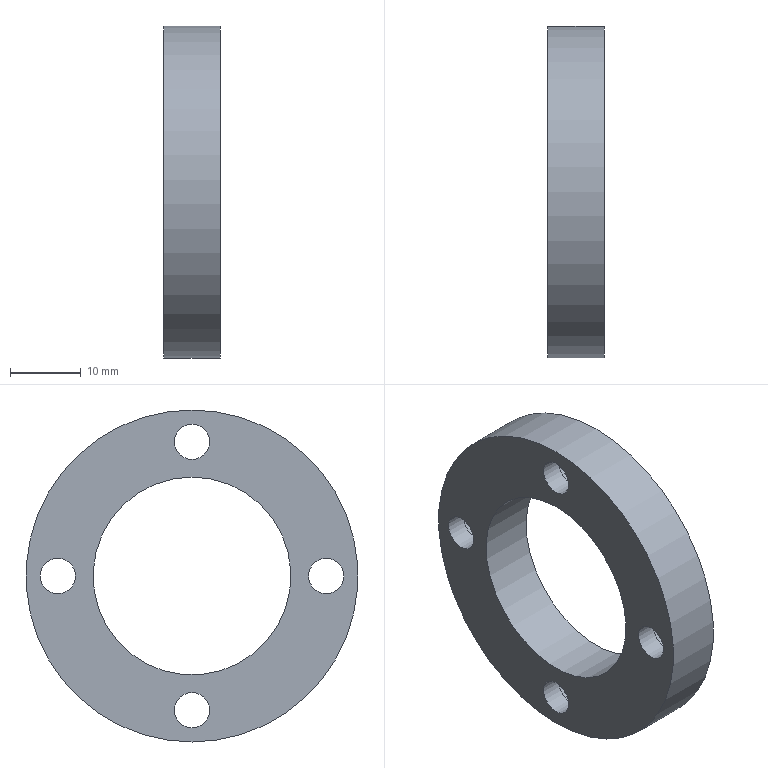Component | NX | SPACER_SLEEVE | 1 solid | 16 faces | box 8 x 47 x 47 mm | volume 7948 mm3 | cylinder 10 | plane 6 | commonest cylinder face diameters 5 x4 7 x4 47 x1 28 x1
STEP:
#1=CARTESIAN_POINT('',(0.,0.,0.));
#2=DIRECTION('',(0.,0.,1.));
#3=DIRECTION('',(1.,0.,0.));
#4=AXIS2_PLACEMENT_3D('',#1,#2,#3);
#5=CARTESIAN_POINT('',(-7.772,-17.527,-244.719));
#6=VERTEX_POINT('',#5);
#7=CARTESIAN_POINT('',(-7.772,-17.527,-258.719));
#8=DIRECTION('',(-1.,0.,0.));
#9=DIRECTION('',(0.,0.,1.));
#10=AXIS2_PLACEMENT_3D('',#7,#8,#9);
#11=CIRCLE('',#10,14.);
#12=CARTESIAN_POINT('',(-7.772,-17.527,-258.719));
#13=DIRECTION('',(1.,0.,0.));
#14=DIRECTION('',(0.,0.,-1.));
#15=AXIS2_PLACEMENT_3D('',#12,#13,#14);
#16=PLANE('',#15);
#17=CARTESIAN_POINT('',(-14.,0.));
#18=CARTESIAN_POINT('',(-14.,24.249));
#19=CARTESIAN_POINT('',(7.,12.124));
#20=CARTESIAN_POINT('',(28.,0.));
#21=CARTESIAN_POINT('',(7.,-12.124));
#22=CARTESIAN_POINT('',(-14.,-24.249));
#23=CARTESIAN_POINT('',(-14.,0.));
#24=(BOUNDED_CURVE()B_SPLINE_CURVE(2,(#17,#18,#19,#20,#21,#22,#23),.UNSPECIFIED.,.T.,.F.)B_SPLINE_CURVE_WITH_KNOTS((1,2,2,2,2,1),(-2.094,0.,2.094,4.189,6.283,8.378),.UNSPECIFIED.)CURVE()GEOMETRIC_REPRESENTATION_ITEM()RATIONAL_B_SPLINE_CURVE((1.,0.5,1.,0.5,1.,0.5,1.))REPRESENTATION_ITEM(''));
#25=(GEOMETRIC_REPRESENTATION_CONTEXT(2)PARAMETRIC_REPRESENTATION_CONTEXT()REPRESENTATION_CONTEXT('',''));
#26=DEFINITIONAL_REPRESENTATION('',(#24),#25);
#27=PCURVE('',#16,#26);
#28=CARTESIAN_POINT('',(-7.772,-17.527,-258.719));
#29=DIRECTION('',(-1.,0.,0.));
#30=DIRECTION('',(0.,0.,1.));
#31=AXIS2_PLACEMENT_3D('',#28,#29,#30);
#32=CYLINDRICAL_SURFACE('',#31,14.);
#33=CARTESIAN_POINT('',(0.,0.));
#34=DIRECTION('',(1.,0.));
#35=VECTOR('',#34,1.);
#36=LINE('',#33,#35);
#37=(GEOMETRIC_REPRESENTATION_CONTEXT(2)PARAMETRIC_REPRESENTATION_CONTEXT()REPRESENTATION_CONTEXT('',''));
#38=DEFINITIONAL_REPRESENTATION('',(#36),#37);
#39=PCURVE('',#32,#38);
#40=SURFACE_CURVE('',#11,(#27,#39),.PCURVE_S1.);
#41=EDGE_CURVE('',#6,#6,#40,.T.);
#42=ORIENTED_EDGE('',*,*,#41,.T.);
#43=EDGE_LOOP('',(#42));
#44=FACE_BOUND('',#43,.T.);
#45=CARTESIAN_POINT('',(-7.772,-17.527,-274.219));
#46=VERTEX_POINT('',#45);
#47=CARTESIAN_POINT('',(-7.772,-17.527,-277.719));
#48=DIRECTION('',(-1.,0.,0.));
#49=DIRECTION('',(0.,0.,1.));
#50=AXIS2_PLACEMENT_3D('',#47,#48,#49);
#51=CIRCLE('',#50,3.5);
#52=CARTESIAN_POINT('',(15.5,-0.));
#53=CARTESIAN_POINT('',(15.5,6.062));
#54=CARTESIAN_POINT('',(20.75,3.031));
#55=CARTESIAN_POINT('',(26.,-0.));
#56=CARTESIAN_POINT('',(20.75,-3.031));
#57=CARTESIAN_POINT('',(15.5,-6.062));
#58=CARTESIAN_POINT('',(15.5,-0.));
#59=(BOUNDED_CURVE()B_SPLINE_CURVE(2,(#52,#53,#54,#55,#56,#57,#58),.UNSPECIFIED.,.T.,.F.)B_SPLINE_CURVE_WITH_KNOTS((1,2,2,2,2,1),(-2.094,0.,2.094,4.189,6.283,8.378),.UNSPECIFIED.)CURVE()GEOMETRIC_REPRESENTATION_ITEM()RATIONAL_B_SPLINE_CURVE((1.,0.5,1.,0.5,1.,0.5,1.))REPRESENTATION_ITEM(''));
#60=(GEOMETRIC_REPRESENTATION_CONTEXT(2)PARAMETRIC_REPRESENTATION_CONTEXT()REPRESENTATION_CONTEXT('',''));
#61=DEFINITIONAL_REPRESENTATION('',(#59),#60);
#62=PCURVE('',#16,#61);
#63=CARTESIAN_POINT('',(-7.772,-17.527,-277.719));
#64=DIRECTION('',(-1.,0.,0.));
#65=DIRECTION('',(0.,0.,1.));
#66=AXIS2_PLACEMENT_3D('',#63,#64,#65);
#67=CYLINDRICAL_SURFACE('',#66,3.5);
#68=CARTESIAN_POINT('',(0.,0.));
#69=DIRECTION('',(1.,0.));
#70=VECTOR('',#69,1.);
#71=LINE('',#68,#70);
#72=(GEOMETRIC_REPRESENTATION_CONTEXT(2)PARAMETRIC_REPRESENTATION_CONTEXT()REPRESENTATION_CONTEXT('',''));
#73=DEFINITIONAL_REPRESENTATION('',(#71),#72);
#74=PCURVE('',#67,#73);
#75=SURFACE_CURVE('',#51,(#62,#74),.PCURVE_S1.);
#76=EDGE_CURVE('',#46,#46,#75,.T.);
#77=ORIENTED_EDGE('',*,*,#76,.T.);
#78=EDGE_LOOP('',(#77));
#79=FACE_BOUND('',#78,.T.);
#80=CARTESIAN_POINT('',(-7.772,-36.527,-255.219));
#81=VERTEX_POINT('',#80);
#82=CARTESIAN_POINT('',(-7.772,-36.527,-258.719));
#83=DIRECTION('',(-1.,0.,0.));
#84=DIRECTION('',(0.,0.,1.));
#85=AXIS2_PLACEMENT_3D('',#82,#83,#84);
#86=CIRCLE('',#85,3.5);
#87=CARTESIAN_POINT('',(-3.5,-19.));
#88=CARTESIAN_POINT('',(-3.5,-12.938));
#89=CARTESIAN_POINT('',(1.75,-15.969));
#90=CARTESIAN_POINT('',(7.,-19.));
#91=CARTESIAN_POINT('',(1.75,-22.031));
#92=CARTESIAN_POINT('',(-3.5,-25.062));
#93=CARTESIAN_POINT('',(-3.5,-19.));
#94=(BOUNDED_CURVE()B_SPLINE_CURVE(2,(#87,#88,#89,#90,#91,#92,#93),.UNSPECIFIED.,.T.,.F.)B_SPLINE_CURVE_WITH_KNOTS((1,2,2,2,2,1),(-2.094,0.,2.094,4.189,6.283,8.378),.UNSPECIFIED.)CURVE()GEOMETRIC_REPRESENTATION_ITEM()RATIONAL_B_SPLINE_CURVE((1.,0.5,1.,0.5,1.,0.5,1.))REPRESENTATION_ITEM(''));
#95=(GEOMETRIC_REPRESENTATION_CONTEXT(2)PARAMETRIC_REPRESENTATION_CONTEXT()REPRESENTATION_CONTEXT('',''));
#96=DEFINITIONAL_REPRESENTATION('',(#94),#95);
#97=PCURVE('',#16,#96);
#98=CARTESIAN_POINT('',(-7.772,-36.527,-258.719));
#99=DIRECTION('',(-1.,0.,0.));
#100=DIRECTION('',(0.,0.,1.));
#101=AXIS2_PLACEMENT_3D('',#98,#99,#100);
#102=CYLINDRICAL_SURFACE('',#101,3.5);
#103=CARTESIAN_POINT('',(0.,0.));
#104=DIRECTION('',(1.,0.));
#105=VECTOR('',#104,1.);
#106=LINE('',#103,#105);
#107=(GEOMETRIC_REPRESENTATION_CONTEXT(2)PARAMETRIC_REPRESENTATION_CONTEXT()REPRESENTATION_CONTEXT('',''));
#108=DEFINITIONAL_REPRESENTATION('',(#106),#107);
#109=PCURVE('',#102,#108);
#110=SURFACE_CURVE('',#86,(#97,#109),.PCURVE_S1.);
#111=EDGE_CURVE('',#81,#81,#110,.T.);
#112=ORIENTED_EDGE('',*,*,#111,.T.);
#113=EDGE_LOOP('',(#112));
#114=FACE_BOUND('',#113,.T.);
#115=CARTESIAN_POINT('',(-7.772,-17.527,-236.219));
#116=VERTEX_POINT('',#115);
#117=CARTESIAN_POINT('',(-7.772,-17.527,-239.719));
#118=DIRECTION('',(-1.,0.,0.));
#119=DIRECTION('',(0.,0.,1.));
#120=AXIS2_PLACEMENT_3D('',#117,#118,#119);
#121=CIRCLE('',#120,3.5);
#122=CARTESIAN_POINT('',(-22.5,0.));
#123=CARTESIAN_POINT('',(-22.5,6.062));
#124=CARTESIAN_POINT('',(-17.25,3.031));
#125=CARTESIAN_POINT('',(-12.,0.));
#126=CARTESIAN_POINT('',(-17.25,-3.031));
#127=CARTESIAN_POINT('',(-22.5,-6.062));
#128=CARTESIAN_POINT('',(-22.5,0.));
#129=(BOUNDED_CURVE()B_SPLINE_CURVE(2,(#122,#123,#124,#125,#126,#127,#128),.UNSPECIFIED.,.T.,.F.)B_SPLINE_CURVE_WITH_KNOTS((1,2,2,2,2,1),(-2.094,0.,2.094,4.189,6.283,8.378),.UNSPECIFIED.)CURVE()GEOMETRIC_REPRESENTATION_ITEM()RATIONAL_B_SPLINE_CURVE((1.,0.5,1.,0.5,1.,0.5,1.))REPRESENTATION_ITEM(''));
#130=(GEOMETRIC_REPRESENTATION_CONTEXT(2)PARAMETRIC_REPRESENTATION_CONTEXT()REPRESENTATION_CONTEXT('',''));
#131=DEFINITIONAL_REPRESENTATION('',(#129),#130);
#132=PCURVE('',#16,#131);
#133=CARTESIAN_POINT('',(-7.772,-17.527,-239.719));
#134=DIRECTION('',(-1.,0.,0.));
#135=DIRECTION('',(0.,0.,1.));
#136=AXIS2_PLACEMENT_3D('',#133,#134,#135);
#137=CYLINDRICAL_SURFACE('',#136,3.5);
#138=CARTESIAN_POINT('',(0.,0.));
#139=DIRECTION('',(1.,0.));
#140=VECTOR('',#139,1.);
#141=LINE('',#138,#140);
#142=(GEOMETRIC_REPRESENTATION_CONTEXT(2)PARAMETRIC_REPRESENTATION_CONTEXT()REPRESENTATION_CONTEXT('',''));
#143=DEFINITIONAL_REPRESENTATION('',(#141),#142);
#144=PCURVE('',#137,#143);
#145=SURFACE_CURVE('',#121,(#132,#144),.PCURVE_S1.);
#146=EDGE_CURVE('',#116,#116,#145,.T.);
#147=ORIENTED_EDGE('',*,*,#146,.T.);
#148=EDGE_LOOP('',(#147));
#149=FACE_BOUND('',#148,.T.);
#150=CARTESIAN_POINT('',(-7.772,1.473,-255.219));
#151=VERTEX_POINT('',#150);
#152=CARTESIAN_POINT('',(-7.772,1.473,-258.719));
#153=DIRECTION('',(-1.,0.,0.));
#154=DIRECTION('',(0.,0.,1.));
#155=AXIS2_PLACEMENT_3D('',#152,#153,#154);
#156=CIRCLE('',#155,3.5);
#157=CARTESIAN_POINT('',(-3.5,19.));
#158=CARTESIAN_POINT('',(-3.5,25.062));
#159=CARTESIAN_POINT('',(1.75,22.031));
#160=CARTESIAN_POINT('',(7.,19.));
#161=CARTESIAN_POINT('',(1.75,15.969));
#162=CARTESIAN_POINT('',(-3.5,12.938));
#163=CARTESIAN_POINT('',(-3.5,19.));
#164=(BOUNDED_CURVE()B_SPLINE_CURVE(2,(#157,#158,#159,#160,#161,#162,#163),.UNSPECIFIED.,.T.,.F.)B_SPLINE_CURVE_WITH_KNOTS((1,2,2,2,2,1),(-2.094,0.,2.094,4.189,6.283,8.378),.UNSPECIFIED.)CURVE()GEOMETRIC_REPRESENTATION_ITEM()RATIONAL_B_SPLINE_CURVE((1.,0.5,1.,0.5,1.,0.5,1.))REPRESENTATION_ITEM(''));
#165=(GEOMETRIC_REPRESENTATION_CONTEXT(2)PARAMETRIC_REPRESENTATION_CONTEXT()REPRESENTATION_CONTEXT('',''));
#166=DEFINITIONAL_REPRESENTATION('',(#164),#165);
#167=PCURVE('',#16,#166);
#168=CARTESIAN_POINT('',(-7.772,1.473,-258.719));
#169=DIRECTION('',(-1.,0.,0.));
#170=DIRECTION('',(0.,0.,1.));
#171=AXIS2_PLACEMENT_3D('',#168,#169,#170);
#172=CYLINDRICAL_SURFACE('',#171,3.5);
#173=CARTESIAN_POINT('',(0.,0.));
#174=DIRECTION('',(1.,0.));
#175=VECTOR('',#174,1.);
#176=LINE('',#173,#175);
#177=(GEOMETRIC_REPRESENTATION_CONTEXT(2)PARAMETRIC_REPRESENTATION_CONTEXT()REPRESENTATION_CONTEXT('',''));
#178=DEFINITIONAL_REPRESENTATION('',(#176),#177);
#179=PCURVE('',#172,#178);
#180=SURFACE_CURVE('',#156,(#167,#179),.PCURVE_S1.);
#181=EDGE_CURVE('',#151,#151,#180,.T.);
#182=ORIENTED_EDGE('',*,*,#181,.T.);
#183=EDGE_LOOP('',(#182));
#184=FACE_BOUND('',#183,.T.);
#185=CARTESIAN_POINT('',(-7.772,-17.527,-282.219));
#186=VERTEX_POINT('',#185);
#187=CARTESIAN_POINT('',(-7.772,-17.527,-258.719));
#188=DIRECTION('',(-1.,0.,0.));
#189=DIRECTION('',(0.,0.,-1.));
#190=AXIS2_PLACEMENT_3D('',#187,#188,#189);
#191=CIRCLE('',#190,23.5);
#192=CARTESIAN_POINT('',(23.5,0.));
#193=CARTESIAN_POINT('',(23.5,-40.703));
#194=CARTESIAN_POINT('',(-11.75,-20.352));
#195=CARTESIAN_POINT('',(-47.,-0.));
#196=CARTESIAN_POINT('',(-11.75,20.352));
#197=CARTESIAN_POINT('',(23.5,40.703));
#198=CARTESIAN_POINT('',(23.5,0.));
#199=(BOUNDED_CURVE()B_SPLINE_CURVE(2,(#192,#193,#194,#195,#196,#197,#198),.UNSPECIFIED.,.T.,.F.)B_SPLINE_CURVE_WITH_KNOTS((1,2,2,2,2,1),(-2.094,0.,2.094,4.189,6.283,8.378),.UNSPECIFIED.)CURVE()GEOMETRIC_REPRESENTATION_ITEM()RATIONAL_B_SPLINE_CURVE((1.,0.5,1.,0.5,1.,0.5,1.))REPRESENTATION_ITEM(''));
#200=(GEOMETRIC_REPRESENTATION_CONTEXT(2)PARAMETRIC_REPRESENTATION_CONTEXT()REPRESENTATION_CONTEXT('',''));
#201=DEFINITIONAL_REPRESENTATION('',(#199),#200);
#202=PCURVE('',#16,#201);
#203=CARTESIAN_POINT('',(-15.772,-17.527,-258.719));
#204=DIRECTION('',(1.,0.,0.));
#205=DIRECTION('',(0.,0.,-1.));
#206=AXIS2_PLACEMENT_3D('',#203,#204,#205);
#207=CYLINDRICAL_SURFACE('',#206,23.5);
#208=CARTESIAN_POINT('',(6.283,8.));
#209=DIRECTION('',(-1.,0.));
#210=VECTOR('',#209,1.);
#211=LINE('',#208,#210);
#212=(GEOMETRIC_REPRESENTATION_CONTEXT(2)PARAMETRIC_REPRESENTATION_CONTEXT()REPRESENTATION_CONTEXT('',''));
#213=DEFINITIONAL_REPRESENTATION('',(#211),#212);
#214=PCURVE('',#207,#213);
#215=SURFACE_CURVE('',#191,(#202,#214),.PCURVE_S1.);
#216=EDGE_CURVE('',#186,#186,#215,.T.);
#217=ORIENTED_EDGE('',*,*,#216,.F.);
#218=EDGE_LOOP('',(#217));
#219=FACE_BOUND('',#218,.T.);
#220=ADVANCED_FACE('',(#44,#79,#114,#149,#184,#219),#16,.T.);
#221=CARTESIAN_POINT('',(-15.772,-17.527,-244.719));
#222=VERTEX_POINT('',#221);
#223=CARTESIAN_POINT('',(-15.772,-17.527,-258.719));
#224=DIRECTION('',(-1.,0.,0.));
#225=DIRECTION('',(0.,0.,1.));
#226=AXIS2_PLACEMENT_3D('',#223,#224,#225);
#227=CIRCLE('',#226,14.);
#228=CARTESIAN_POINT('',(-15.772,-17.527,-258.719));
#229=DIRECTION('',(-1.,0.,0.));
#230=DIRECTION('',(0.,0.,1.));
#231=AXIS2_PLACEMENT_3D('',#228,#229,#230);
#232=PLANE('',#231);
#233=CARTESIAN_POINT('',(0.,0.));
#234=DIRECTION('',(1.,0.));
#235=AXIS2_PLACEMENT_2D('',#233,#234);
#236=CIRCLE('',#235,14.);
#237=(GEOMETRIC_REPRESENTATION_CONTEXT(2)PARAMETRIC_REPRESENTATION_CONTEXT()REPRESENTATION_CONTEXT('',''));
#238=DEFINITIONAL_REPRESENTATION('',(#236),#237);
#239=PCURVE('',#232,#238);
#240=CARTESIAN_POINT('',(0.,8.));
#241=DIRECTION('',(1.,0.));
#242=VECTOR('',#241,1.);
#243=LINE('',#240,#242);
#244=(GEOMETRIC_REPRESENTATION_CONTEXT(2)PARAMETRIC_REPRESENTATION_CONTEXT()REPRESENTATION_CONTEXT('',''));
#245=DEFINITIONAL_REPRESENTATION('',(#243),#244);
#246=PCURVE('',#32,#245);
#247=SURFACE_CURVE('',#227,(#239,#246),.PCURVE_S1.);
#248=EDGE_CURVE('',#222,#222,#247,.T.);
#249=ORIENTED_EDGE('',*,*,#248,.F.);
#250=EDGE_LOOP('',(#249));
#251=FACE_BOUND('',#250,.T.);
#252=CARTESIAN_POINT('',(-15.772,-17.527,-275.219));
#253=VERTEX_POINT('',#252);
#254=CARTESIAN_POINT('',(-15.772,-17.527,-277.719));
#255=DIRECTION('',(-1.,0.,0.));
#256=DIRECTION('',(0.,0.,1.));
#257=AXIS2_PLACEMENT_3D('',#254,#255,#256);
#258=CIRCLE('',#257,2.5);
#259=CARTESIAN_POINT('',(-19.,-0.));
#260=DIRECTION('',(1.,0.));
#261=AXIS2_PLACEMENT_2D('',#259,#260);
#262=CIRCLE('',#261,2.5);
#263=(GEOMETRIC_REPRESENTATION_CONTEXT(2)PARAMETRIC_REPRESENTATION_CONTEXT()REPRESENTATION_CONTEXT('',''));
#264=DEFINITIONAL_REPRESENTATION('',(#262),#263);
#265=PCURVE('',#232,#264);
#266=CARTESIAN_POINT('',(-43.312,-17.527,-277.719));
#267=DIRECTION('',(-1.,0.,0.));
#268=DIRECTION('',(0.,0.,1.));
#269=AXIS2_PLACEMENT_3D('',#266,#267,#268);
#270=CYLINDRICAL_SURFACE('',#269,2.5);
#271=CARTESIAN_POINT('',(0.,-27.541));
#272=DIRECTION('',(1.,0.));
#273=VECTOR('',#272,1.);
#274=LINE('',#271,#273);
#275=(GEOMETRIC_REPRESENTATION_CONTEXT(2)PARAMETRIC_REPRESENTATION_CONTEXT()REPRESENTATION_CONTEXT('',''));
#276=DEFINITIONAL_REPRESENTATION('',(#274),#275);
#277=PCURVE('',#270,#276);
#278=SURFACE_CURVE('',#258,(#265,#277),.PCURVE_S1.);
#279=EDGE_CURVE('',#253,#253,#278,.T.);
#280=ORIENTED_EDGE('',*,*,#279,.F.);
#281=EDGE_LOOP('',(#280));
#282=FACE_BOUND('',#281,.T.);
#283=CARTESIAN_POINT('',(-15.772,-36.527,-256.219));
#284=VERTEX_POINT('',#283);
#285=CARTESIAN_POINT('',(-15.772,-36.527,-258.719));
#286=DIRECTION('',(-1.,0.,0.));
#287=DIRECTION('',(0.,0.,1.));
#288=AXIS2_PLACEMENT_3D('',#285,#286,#287);
#289=CIRCLE('',#288,2.5);
#290=CARTESIAN_POINT('',(0.,-19.));
#291=DIRECTION('',(1.,0.));
#292=AXIS2_PLACEMENT_2D('',#290,#291);
#293=CIRCLE('',#292,2.5);
#294=(GEOMETRIC_REPRESENTATION_CONTEXT(2)PARAMETRIC_REPRESENTATION_CONTEXT()REPRESENTATION_CONTEXT('',''));
#295=DEFINITIONAL_REPRESENTATION('',(#293),#294);
#296=PCURVE('',#232,#295);
#297=CARTESIAN_POINT('',(-43.312,-36.527,-258.719));
#298=DIRECTION('',(-1.,0.,0.));
#299=DIRECTION('',(0.,0.,1.));
#300=AXIS2_PLACEMENT_3D('',#297,#298,#299);
#301=CYLINDRICAL_SURFACE('',#300,2.5);
#302=CARTESIAN_POINT('',(0.,-27.541));
#303=DIRECTION('',(1.,0.));
#304=VECTOR('',#303,1.);
#305=LINE('',#302,#304);
#306=(GEOMETRIC_REPRESENTATION_CONTEXT(2)PARAMETRIC_REPRESENTATION_CONTEXT()REPRESENTATION_CONTEXT('',''));
#307=DEFINITIONAL_REPRESENTATION('',(#305),#306);
#308=PCURVE('',#301,#307);
#309=SURFACE_CURVE('',#289,(#296,#308),.PCURVE_S1.);
#310=EDGE_CURVE('',#284,#284,#309,.T.);
#311=ORIENTED_EDGE('',*,*,#310,.F.);
#312=EDGE_LOOP('',(#311));
#313=FACE_BOUND('',#312,.T.);
#314=CARTESIAN_POINT('',(-15.772,-17.527,-237.219));
#315=VERTEX_POINT('',#314);
#316=CARTESIAN_POINT('',(-15.772,-17.527,-239.719));
#317=DIRECTION('',(-1.,0.,0.));
#318=DIRECTION('',(0.,0.,1.));
#319=AXIS2_PLACEMENT_3D('',#316,#317,#318);
#320=CIRCLE('',#319,2.5);
#321=CARTESIAN_POINT('',(19.,0.));
#322=DIRECTION('',(1.,0.));
#323=AXIS2_PLACEMENT_2D('',#321,#322);
#324=CIRCLE('',#323,2.5);
#325=(GEOMETRIC_REPRESENTATION_CONTEXT(2)PARAMETRIC_REPRESENTATION_CONTEXT()REPRESENTATION_CONTEXT('',''));
#326=DEFINITIONAL_REPRESENTATION('',(#324),#325);
#327=PCURVE('',#232,#326);
#328=CARTESIAN_POINT('',(-43.312,-17.527,-239.719));
#329=DIRECTION('',(-1.,0.,0.));
#330=DIRECTION('',(0.,0.,1.));
#331=AXIS2_PLACEMENT_3D('',#328,#329,#330);
#332=CYLINDRICAL_SURFACE('',#331,2.5);
#333=CARTESIAN_POINT('',(0.,-27.541));
#334=DIRECTION('',(1.,0.));
#335=VECTOR('',#334,1.);
#336=LINE('',#333,#335);
#337=(GEOMETRIC_REPRESENTATION_CONTEXT(2)PARAMETRIC_REPRESENTATION_CONTEXT()REPRESENTATION_CONTEXT('',''));
#338=DEFINITIONAL_REPRESENTATION('',(#336),#337);
#339=PCURVE('',#332,#338);
#340=SURFACE_CURVE('',#320,(#327,#339),.PCURVE_S1.);
#341=EDGE_CURVE('',#315,#315,#340,.T.);
#342=ORIENTED_EDGE('',*,*,#341,.F.);
#343=EDGE_LOOP('',(#342));
#344=FACE_BOUND('',#343,.T.);
#345=CARTESIAN_POINT('',(-15.772,1.473,-256.219));
#346=VERTEX_POINT('',#345);
#347=CARTESIAN_POINT('',(-15.772,1.473,-258.719));
#348=DIRECTION('',(-1.,0.,0.));
#349=DIRECTION('',(0.,0.,1.));
#350=AXIS2_PLACEMENT_3D('',#347,#348,#349);
#351=CIRCLE('',#350,2.5);
#352=CARTESIAN_POINT('',(-0.,19.));
#353=DIRECTION('',(1.,0.));
#354=AXIS2_PLACEMENT_2D('',#352,#353);
#355=CIRCLE('',#354,2.5);
#356=(GEOMETRIC_REPRESENTATION_CONTEXT(2)PARAMETRIC_REPRESENTATION_CONTEXT()REPRESENTATION_CONTEXT('',''));
#357=DEFINITIONAL_REPRESENTATION('',(#355),#356);
#358=PCURVE('',#232,#357);
#359=CARTESIAN_POINT('',(-43.312,1.473,-258.719));
#360=DIRECTION('',(-1.,0.,0.));
#361=DIRECTION('',(0.,0.,1.));
#362=AXIS2_PLACEMENT_3D('',#359,#360,#361);
#363=CYLINDRICAL_SURFACE('',#362,2.5);
#364=CARTESIAN_POINT('',(0.,-27.541));
#365=DIRECTION('',(1.,0.));
#366=VECTOR('',#365,1.);
#367=LINE('',#364,#366);
#368=(GEOMETRIC_REPRESENTATION_CONTEXT(2)PARAMETRIC_REPRESENTATION_CONTEXT()REPRESENTATION_CONTEXT('',''));
#369=DEFINITIONAL_REPRESENTATION('',(#367),#368);
#370=PCURVE('',#363,#369);
#371=SURFACE_CURVE('',#351,(#358,#370),.PCURVE_S1.);
#372=EDGE_CURVE('',#346,#346,#371,.T.);
#373=ORIENTED_EDGE('',*,*,#372,.F.);
#374=EDGE_LOOP('',(#373));
#375=FACE_BOUND('',#374,.T.);
#376=CARTESIAN_POINT('',(-15.772,-17.527,-282.219));
#377=VERTEX_POINT('',#376);
#378=CARTESIAN_POINT('',(-15.772,-17.527,-258.719));
#379=DIRECTION('',(1.,0.,0.));
#380=DIRECTION('',(0.,0.,-1.));
#381=AXIS2_PLACEMENT_3D('',#378,#379,#380);
#382=CIRCLE('',#381,23.5);
#383=CARTESIAN_POINT('',(-23.5,0.));
#384=CARTESIAN_POINT('',(-23.5,40.703));
#385=CARTESIAN_POINT('',(11.75,20.352));
#386=CARTESIAN_POINT('',(47.,0.));
#387=CARTESIAN_POINT('',(11.75,-20.352));
#388=CARTESIAN_POINT('',(-23.5,-40.703));
#389=CARTESIAN_POINT('',(-23.5,0.));
#390=(BOUNDED_CURVE()B_SPLINE_CURVE(2,(#383,#384,#385,#386,#387,#388,#389),.UNSPECIFIED.,.T.,.F.)B_SPLINE_CURVE_WITH_KNOTS((1,2,2,2,2,1),(-2.094,0.,2.094,4.189,6.283,8.378),.UNSPECIFIED.)CURVE()GEOMETRIC_REPRESENTATION_ITEM()RATIONAL_B_SPLINE_CURVE((1.,0.5,1.,0.5,1.,0.5,1.))REPRESENTATION_ITEM(''));
#391=(GEOMETRIC_REPRESENTATION_CONTEXT(2)PARAMETRIC_REPRESENTATION_CONTEXT()REPRESENTATION_CONTEXT('',''));
#392=DEFINITIONAL_REPRESENTATION('',(#390),#391);
#393=PCURVE('',#232,#392);
#394=CARTESIAN_POINT('',(0.,0.));
#395=DIRECTION('',(1.,0.));
#396=VECTOR('',#395,1.);
#397=LINE('',#394,#396);
#398=(GEOMETRIC_REPRESENTATION_CONTEXT(2)PARAMETRIC_REPRESENTATION_CONTEXT()REPRESENTATION_CONTEXT('',''));
#399=DEFINITIONAL_REPRESENTATION('',(#397),#398);
#400=PCURVE('',#207,#399);
#401=SURFACE_CURVE('',#382,(#393,#400),.PCURVE_S1.);
#402=EDGE_CURVE('',#377,#377,#401,.T.);
#403=ORIENTED_EDGE('',*,*,#402,.F.);
#404=EDGE_LOOP('',(#403));
#405=FACE_BOUND('',#404,.T.);
#406=ADVANCED_FACE('',(#251,#282,#313,#344,#375,#405),#232,.T.);
#407=ORIENTED_EDGE('',*,*,#216,.T.);
#408=CARTESIAN_POINT('',(-15.772,-17.527,-282.219));
#409=CARTESIAN_POINT('',(-7.772,-17.527,-282.219));
#410=B_SPLINE_CURVE_WITH_KNOTS('',1,(#408,#409),.UNSPECIFIED.,.F.,.F.,(2,2),(0.,8.),.PIECEWISE_BEZIER_KNOTS.);
#411=CARTESIAN_POINT('',(0.,0.));
#412=DIRECTION('',(0.,1.));
#413=VECTOR('',#412,1.);
#414=LINE('',#411,#413);
#415=(GEOMETRIC_REPRESENTATION_CONTEXT(2)PARAMETRIC_REPRESENTATION_CONTEXT()REPRESENTATION_CONTEXT('',''));
#416=DEFINITIONAL_REPRESENTATION('',(#414),#415);
#417=PCURVE('',#207,#416);
#418=CARTESIAN_POINT('',(6.283,0.));
#419=DIRECTION('',(0.,1.));
#420=VECTOR('',#419,1.);
#421=LINE('',#418,#420);
#422=(GEOMETRIC_REPRESENTATION_CONTEXT(2)PARAMETRIC_REPRESENTATION_CONTEXT()REPRESENTATION_CONTEXT('',''));
#423=DEFINITIONAL_REPRESENTATION('',(#421),#422);
#424=PCURVE('',#207,#423);
#425=SEAM_CURVE('',#410,(#417,#424),.PCURVE_S1.);
#426=EDGE_CURVE('',#377,#186,#425,.T.);
#427=ORIENTED_EDGE('',*,*,#426,.F.);
#428=ORIENTED_EDGE('',*,*,#402,.T.);
#429=ORIENTED_EDGE('',*,*,#426,.T.);
#430=EDGE_LOOP('',(#407,#427,#428,#429));
#431=FACE_BOUND('',#430,.T.);
#432=ADVANCED_FACE('',(#431),#207,.T.);
#433=ORIENTED_EDGE('',*,*,#372,.F.);
#434=CARTESIAN_POINT('',(-12.772,1.473,-256.219));
#435=VERTEX_POINT('',#434);
#436=CARTESIAN_POINT('',(-12.772,1.473,-256.219));
#437=CARTESIAN_POINT('',(-15.772,1.473,-256.219));
#438=B_SPLINE_CURVE_WITH_KNOTS('',1,(#436,#437),.UNSPECIFIED.,.F.,.F.,(2,2),(-30.541,-27.541),.PIECEWISE_BEZIER_KNOTS.);
#439=CARTESIAN_POINT('',(0.,0.));
#440=DIRECTION('',(0.,1.));
#441=VECTOR('',#440,1.);
#442=LINE('',#439,#441);
#443=(GEOMETRIC_REPRESENTATION_CONTEXT(2)PARAMETRIC_REPRESENTATION_CONTEXT()REPRESENTATION_CONTEXT('',''));
#444=DEFINITIONAL_REPRESENTATION('',(#442),#443);
#445=PCURVE('',#363,#444);
#446=CARTESIAN_POINT('',(6.283,0.));
#447=DIRECTION('',(0.,1.));
#448=VECTOR('',#447,1.);
#449=LINE('',#446,#448);
#450=(GEOMETRIC_REPRESENTATION_CONTEXT(2)PARAMETRIC_REPRESENTATION_CONTEXT()REPRESENTATION_CONTEXT('',''));
#451=DEFINITIONAL_REPRESENTATION('',(#449),#450);
#452=PCURVE('',#363,#451);
#453=SEAM_CURVE('',#438,(#445,#452),.PCURVE_S1.);
#454=EDGE_CURVE('',#435,#346,#453,.T.);
#455=ORIENTED_EDGE('',*,*,#454,.F.);
#456=CARTESIAN_POINT('',(-12.772,1.473,-258.719));
#457=DIRECTION('',(1.,0.,0.));
#458=DIRECTION('',(0.,0.,1.));
#459=AXIS2_PLACEMENT_3D('',#456,#457,#458);
#460=CIRCLE('',#459,2.5);
#461=CARTESIAN_POINT('',(6.283,-30.541));
#462=DIRECTION('',(-1.,0.));
#463=VECTOR('',#462,1.);
#464=LINE('',#461,#463);
#465=(GEOMETRIC_REPRESENTATION_CONTEXT(2)PARAMETRIC_REPRESENTATION_CONTEXT()REPRESENTATION_CONTEXT('',''));
#466=DEFINITIONAL_REPRESENTATION('',(#464),#465);
#467=PCURVE('',#363,#466);
#468=CARTESIAN_POINT('',(-12.772,1.473,-258.719));
#469=DIRECTION('',(-1.,0.,0.));
#470=DIRECTION('',(0.,0.,1.));
#471=AXIS2_PLACEMENT_3D('',#468,#469,#470);
#472=PLANE('',#471);
#473=CARTESIAN_POINT('',(2.5,0.));
#474=CARTESIAN_POINT('',(2.5,-4.33));
#475=CARTESIAN_POINT('',(-1.25,-2.165));
#476=CARTESIAN_POINT('',(-5.,-0.));
#477=CARTESIAN_POINT('',(-1.25,2.165));
#478=CARTESIAN_POINT('',(2.5,4.33));
#479=CARTESIAN_POINT('',(2.5,0.));
#480=(BOUNDED_CURVE()B_SPLINE_CURVE(2,(#473,#474,#475,#476,#477,#478,#479),.UNSPECIFIED.,.T.,.F.)B_SPLINE_CURVE_WITH_KNOTS((1,2,2,2,2,1),(-2.094,0.,2.094,4.189,6.283,8.378),.UNSPECIFIED.)CURVE()GEOMETRIC_REPRESENTATION_ITEM()RATIONAL_B_SPLINE_CURVE((1.,0.5,1.,0.5,1.,0.5,1.))REPRESENTATION_ITEM(''));
#481=(GEOMETRIC_REPRESENTATION_CONTEXT(2)PARAMETRIC_REPRESENTATION_CONTEXT()REPRESENTATION_CONTEXT('',''));
#482=DEFINITIONAL_REPRESENTATION('',(#480),#481);
#483=PCURVE('',#472,#482);
#484=SURFACE_CURVE('',#460,(#467,#483),.PCURVE_S1.);
#485=EDGE_CURVE('',#435,#435,#484,.T.);
#486=ORIENTED_EDGE('',*,*,#485,.F.);
#487=ORIENTED_EDGE('',*,*,#454,.T.);
#488=EDGE_LOOP('',(#433,#455,#486,#487));
#489=FACE_BOUND('',#488,.F.);
#490=ADVANCED_FACE('',(#489),#363,.F.);
#491=ORIENTED_EDGE('',*,*,#485,.F.);
#492=EDGE_LOOP('',(#491));
#493=FACE_BOUND('',#492,.T.);
#494=CARTESIAN_POINT('',(-12.772,1.473,-255.219));
#495=VERTEX_POINT('',#494);
#496=CARTESIAN_POINT('',(-12.772,1.473,-258.719));
#497=DIRECTION('',(1.,0.,0.));
#498=DIRECTION('',(0.,0.,1.));
#499=AXIS2_PLACEMENT_3D('',#496,#497,#498);
#500=CIRCLE('',#499,3.5);
#501=CARTESIAN_POINT('',(3.5,0.));
#502=CARTESIAN_POINT('',(3.5,-6.062));
#503=CARTESIAN_POINT('',(-1.75,-3.031));
#504=CARTESIAN_POINT('',(-7.,-0.));
#505=CARTESIAN_POINT('',(-1.75,3.031));
#506=CARTESIAN_POINT('',(3.5,6.062));
#507=CARTESIAN_POINT('',(3.5,0.));
#508=(BOUNDED_CURVE()B_SPLINE_CURVE(2,(#501,#502,#503,#504,#505,#506,#507),.UNSPECIFIED.,.T.,.F.)B_SPLINE_CURVE_WITH_KNOTS((1,2,2,2,2,1),(-2.094,0.,2.094,4.189,6.283,8.378),.UNSPECIFIED.)CURVE()GEOMETRIC_REPRESENTATION_ITEM()RATIONAL_B_SPLINE_CURVE((1.,0.5,1.,0.5,1.,0.5,1.))REPRESENTATION_ITEM(''));
#509=(GEOMETRIC_REPRESENTATION_CONTEXT(2)PARAMETRIC_REPRESENTATION_CONTEXT()REPRESENTATION_CONTEXT('',''));
#510=DEFINITIONAL_REPRESENTATION('',(#508),#509);
#511=PCURVE('',#472,#510);
#512=CARTESIAN_POINT('',(6.283,5.));
#513=DIRECTION('',(-1.,0.));
#514=VECTOR('',#513,1.);
#515=LINE('',#512,#514);
#516=(GEOMETRIC_REPRESENTATION_CONTEXT(2)PARAMETRIC_REPRESENTATION_CONTEXT()REPRESENTATION_CONTEXT('',''));
#517=DEFINITIONAL_REPRESENTATION('',(#515),#516);
#518=PCURVE('',#172,#517);
#519=SURFACE_CURVE('',#500,(#511,#518),.PCURVE_S1.);
#520=EDGE_CURVE('',#495,#495,#519,.T.);
#521=ORIENTED_EDGE('',*,*,#520,.T.);
#522=EDGE_LOOP('',(#521));
#523=FACE_BOUND('',#522,.T.);
#524=ADVANCED_FACE('',(#493,#523),#472,.F.);
#525=ORIENTED_EDGE('',*,*,#520,.T.);
#526=CARTESIAN_POINT('',(-7.772,1.473,-255.219));
#527=CARTESIAN_POINT('',(-12.772,1.473,-255.219));
#528=B_SPLINE_CURVE_WITH_KNOTS('',1,(#526,#527),.UNSPECIFIED.,.F.,.F.,(2,2),(0.,5.),.PIECEWISE_BEZIER_KNOTS.);
#529=CARTESIAN_POINT('',(0.,0.));
#530=DIRECTION('',(0.,1.));
#531=VECTOR('',#530,1.);
#532=LINE('',#529,#531);
#533=(GEOMETRIC_REPRESENTATION_CONTEXT(2)PARAMETRIC_REPRESENTATION_CONTEXT()REPRESENTATION_CONTEXT('',''));
#534=DEFINITIONAL_REPRESENTATION('',(#532),#533);
#535=PCURVE('',#172,#534);
#536=CARTESIAN_POINT('',(6.283,0.));
#537=DIRECTION('',(0.,1.));
#538=VECTOR('',#537,1.);
#539=LINE('',#536,#538);
#540=(GEOMETRIC_REPRESENTATION_CONTEXT(2)PARAMETRIC_REPRESENTATION_CONTEXT()REPRESENTATION_CONTEXT('',''));
#541=DEFINITIONAL_REPRESENTATION('',(#539),#540);
#542=PCURVE('',#172,#541);
#543=SEAM_CURVE('',#528,(#535,#542),.PCURVE_S1.);
#544=EDGE_CURVE('',#151,#495,#543,.T.);
#545=ORIENTED_EDGE('',*,*,#544,.F.);
#546=ORIENTED_EDGE('',*,*,#181,.T.);
#547=ORIENTED_EDGE('',*,*,#544,.T.);
#548=EDGE_LOOP('',(#525,#545,#546,#547));
#549=FACE_BOUND('',#548,.F.);
#550=ADVANCED_FACE('',(#549),#172,.F.);
#551=ORIENTED_EDGE('',*,*,#341,.F.);
#552=CARTESIAN_POINT('',(-12.772,-17.527,-237.219));
#553=VERTEX_POINT('',#552);
#554=CARTESIAN_POINT('',(-12.772,-17.527,-237.219));
#555=CARTESIAN_POINT('',(-15.772,-17.527,-237.219));
#556=B_SPLINE_CURVE_WITH_KNOTS('',1,(#554,#555),.UNSPECIFIED.,.F.,.F.,(2,2),(-30.541,-27.541),.PIECEWISE_BEZIER_KNOTS.);
#557=CARTESIAN_POINT('',(0.,0.));
#558=DIRECTION('',(0.,1.));
#559=VECTOR('',#558,1.);
#560=LINE('',#557,#559);
#561=(GEOMETRIC_REPRESENTATION_CONTEXT(2)PARAMETRIC_REPRESENTATION_CONTEXT()REPRESENTATION_CONTEXT('',''));
#562=DEFINITIONAL_REPRESENTATION('',(#560),#561);
#563=PCURVE('',#332,#562);
#564=CARTESIAN_POINT('',(6.283,0.));
#565=DIRECTION('',(0.,1.));
#566=VECTOR('',#565,1.);
#567=LINE('',#564,#566);
#568=(GEOMETRIC_REPRESENTATION_CONTEXT(2)PARAMETRIC_REPRESENTATION_CONTEXT()REPRESENTATION_CONTEXT('',''));
#569=DEFINITIONAL_REPRESENTATION('',(#567),#568);
#570=PCURVE('',#332,#569);
#571=SEAM_CURVE('',#556,(#563,#570),.PCURVE_S1.);
#572=EDGE_CURVE('',#553,#315,#571,.T.);
#573=ORIENTED_EDGE('',*,*,#572,.F.);
#574=CARTESIAN_POINT('',(-12.772,-17.527,-239.719));
#575=DIRECTION('',(1.,0.,0.));
#576=DIRECTION('',(0.,0.,1.));
#577=AXIS2_PLACEMENT_3D('',#574,#575,#576);
#578=CIRCLE('',#577,2.5);
#579=CARTESIAN_POINT('',(6.283,-30.541));
#580=DIRECTION('',(-1.,0.));
#581=VECTOR('',#580,1.);
#582=LINE('',#579,#581);
#583=(GEOMETRIC_REPRESENTATION_CONTEXT(2)PARAMETRIC_REPRESENTATION_CONTEXT()REPRESENTATION_CONTEXT('',''));
#584=DEFINITIONAL_REPRESENTATION('',(#582),#583);
#585=PCURVE('',#332,#584);
#586=CARTESIAN_POINT('',(-12.772,-17.527,-239.719));
#587=DIRECTION('',(-1.,0.,0.));
#588=DIRECTION('',(0.,0.,1.));
#589=AXIS2_PLACEMENT_3D('',#586,#587,#588);
#590=PLANE('',#589);
#591=CARTESIAN_POINT('',(2.5,0.));
#592=CARTESIAN_POINT('',(2.5,-4.33));
#593=CARTESIAN_POINT('',(-1.25,-2.165));
#594=CARTESIAN_POINT('',(-5.,-0.));
#595=CARTESIAN_POINT('',(-1.25,2.165));
#596=CARTESIAN_POINT('',(2.5,4.33));
#597=CARTESIAN_POINT('',(2.5,0.));
#598=(BOUNDED_CURVE()B_SPLINE_CURVE(2,(#591,#592,#593,#594,#595,#596,#597),.UNSPECIFIED.,.T.,.F.)B_SPLINE_CURVE_WITH_KNOTS((1,2,2,2,2,1),(-2.094,0.,2.094,4.189,6.283,8.378),.UNSPECIFIED.)CURVE()GEOMETRIC_REPRESENTATION_ITEM()RATIONAL_B_SPLINE_CURVE((1.,0.5,1.,0.5,1.,0.5,1.))REPRESENTATION_ITEM(''));
#599=(GEOMETRIC_REPRESENTATION_CONTEXT(2)PARAMETRIC_REPRESENTATION_CONTEXT()REPRESENTATION_CONTEXT('',''));
#600=DEFINITIONAL_REPRESENTATION('',(#598),#599);
#601=PCURVE('',#590,#600);
#602=SURFACE_CURVE('',#578,(#585,#601),.PCURVE_S1.);
#603=EDGE_CURVE('',#553,#553,#602,.T.);
#604=ORIENTED_EDGE('',*,*,#603,.F.);
#605=ORIENTED_EDGE('',*,*,#572,.T.);
#606=EDGE_LOOP('',(#551,#573,#604,#605));
#607=FACE_BOUND('',#606,.F.);
#608=ADVANCED_FACE('',(#607),#332,.F.);
#609=ORIENTED_EDGE('',*,*,#603,.F.);
#610=EDGE_LOOP('',(#609));
#611=FACE_BOUND('',#610,.T.);
#612=CARTESIAN_POINT('',(-12.772,-17.527,-236.219));
#613=VERTEX_POINT('',#612);
#614=CARTESIAN_POINT('',(-12.772,-17.527,-239.719));
#615=DIRECTION('',(1.,0.,0.));
#616=DIRECTION('',(0.,0.,1.));
#617=AXIS2_PLACEMENT_3D('',#614,#615,#616);
#618=CIRCLE('',#617,3.5);
#619=CARTESIAN_POINT('',(3.5,0.));
#620=CARTESIAN_POINT('',(3.5,-6.062));
#621=CARTESIAN_POINT('',(-1.75,-3.031));
#622=CARTESIAN_POINT('',(-7.,-0.));
#623=CARTESIAN_POINT('',(-1.75,3.031));
#624=CARTESIAN_POINT('',(3.5,6.062));
#625=CARTESIAN_POINT('',(3.5,0.));
#626=(BOUNDED_CURVE()B_SPLINE_CURVE(2,(#619,#620,#621,#622,#623,#624,#625),.UNSPECIFIED.,.T.,.F.)B_SPLINE_CURVE_WITH_KNOTS((1,2,2,2,2,1),(-2.094,0.,2.094,4.189,6.283,8.378),.UNSPECIFIED.)CURVE()GEOMETRIC_REPRESENTATION_ITEM()RATIONAL_B_SPLINE_CURVE((1.,0.5,1.,0.5,1.,0.5,1.))REPRESENTATION_ITEM(''));
#627=(GEOMETRIC_REPRESENTATION_CONTEXT(2)PARAMETRIC_REPRESENTATION_CONTEXT()REPRESENTATION_CONTEXT('',''));
#628=DEFINITIONAL_REPRESENTATION('',(#626),#627);
#629=PCURVE('',#590,#628);
#630=CARTESIAN_POINT('',(6.283,5.));
#631=DIRECTION('',(-1.,0.));
#632=VECTOR('',#631,1.);
#633=LINE('',#630,#632);
#634=(GEOMETRIC_REPRESENTATION_CONTEXT(2)PARAMETRIC_REPRESENTATION_CONTEXT()REPRESENTATION_CONTEXT('',''));
#635=DEFINITIONAL_REPRESENTATION('',(#633),#634);
#636=PCURVE('',#137,#635);
#637=SURFACE_CURVE('',#618,(#629,#636),.PCURVE_S1.);
#638=EDGE_CURVE('',#613,#613,#637,.T.);
#639=ORIENTED_EDGE('',*,*,#638,.T.);
#640=EDGE_LOOP('',(#639));
#641=FACE_BOUND('',#640,.T.);
#642=ADVANCED_FACE('',(#611,#641),#590,.F.);
#643=ORIENTED_EDGE('',*,*,#638,.T.);
#644=CARTESIAN_POINT('',(-7.772,-17.527,-236.219));
#645=CARTESIAN_POINT('',(-12.772,-17.527,-236.219));
#646=B_SPLINE_CURVE_WITH_KNOTS('',1,(#644,#645),.UNSPECIFIED.,.F.,.F.,(2,2),(0.,5.),.PIECEWISE_BEZIER_KNOTS.);
#647=CARTESIAN_POINT('',(0.,0.));
#648=DIRECTION('',(0.,1.));
#649=VECTOR('',#648,1.);
#650=LINE('',#647,#649);
#651=(GEOMETRIC_REPRESENTATION_CONTEXT(2)PARAMETRIC_REPRESENTATION_CONTEXT()REPRESENTATION_CONTEXT('',''));
#652=DEFINITIONAL_REPRESENTATION('',(#650),#651);
#653=PCURVE('',#137,#652);
#654=CARTESIAN_POINT('',(6.283,0.));
#655=DIRECTION('',(0.,1.));
#656=VECTOR('',#655,1.);
#657=LINE('',#654,#656);
#658=(GEOMETRIC_REPRESENTATION_CONTEXT(2)PARAMETRIC_REPRESENTATION_CONTEXT()REPRESENTATION_CONTEXT('',''));
#659=DEFINITIONAL_REPRESENTATION('',(#657),#658);
#660=PCURVE('',#137,#659);
#661=SEAM_CURVE('',#646,(#653,#660),.PCURVE_S1.);
#662=EDGE_CURVE('',#116,#613,#661,.T.);
#663=ORIENTED_EDGE('',*,*,#662,.F.);
#664=ORIENTED_EDGE('',*,*,#146,.T.);
#665=ORIENTED_EDGE('',*,*,#662,.T.);
#666=EDGE_LOOP('',(#643,#663,#664,#665));
#667=FACE_BOUND('',#666,.F.);
#668=ADVANCED_FACE('',(#667),#137,.F.);
#669=ORIENTED_EDGE('',*,*,#310,.F.);
#670=CARTESIAN_POINT('',(-12.772,-36.527,-256.219));
#671=VERTEX_POINT('',#670);
#672=CARTESIAN_POINT('',(-12.772,-36.527,-256.219));
#673=CARTESIAN_POINT('',(-15.772,-36.527,-256.219));
#674=B_SPLINE_CURVE_WITH_KNOTS('',1,(#672,#673),.UNSPECIFIED.,.F.,.F.,(2,2),(-30.541,-27.541),.PIECEWISE_BEZIER_KNOTS.);
#675=CARTESIAN_POINT('',(0.,0.));
#676=DIRECTION('',(0.,1.));
#677=VECTOR('',#676,1.);
#678=LINE('',#675,#677);
#679=(GEOMETRIC_REPRESENTATION_CONTEXT(2)PARAMETRIC_REPRESENTATION_CONTEXT()REPRESENTATION_CONTEXT('',''));
#680=DEFINITIONAL_REPRESENTATION('',(#678),#679);
#681=PCURVE('',#301,#680);
#682=CARTESIAN_POINT('',(6.283,0.));
#683=DIRECTION('',(0.,1.));
#684=VECTOR('',#683,1.);
#685=LINE('',#682,#684);
#686=(GEOMETRIC_REPRESENTATION_CONTEXT(2)PARAMETRIC_REPRESENTATION_CONTEXT()REPRESENTATION_CONTEXT('',''));
#687=DEFINITIONAL_REPRESENTATION('',(#685),#686);
#688=PCURVE('',#301,#687);
#689=SEAM_CURVE('',#674,(#681,#688),.PCURVE_S1.);
#690=EDGE_CURVE('',#671,#284,#689,.T.);
#691=ORIENTED_EDGE('',*,*,#690,.F.);
#692=CARTESIAN_POINT('',(-12.772,-36.527,-258.719));
#693=DIRECTION('',(1.,0.,0.));
#694=DIRECTION('',(0.,0.,1.));
#695=AXIS2_PLACEMENT_3D('',#692,#693,#694);
#696=CIRCLE('',#695,2.5);
#697=CARTESIAN_POINT('',(6.283,-30.541));
#698=DIRECTION('',(-1.,0.));
#699=VECTOR('',#698,1.);
#700=LINE('',#697,#699);
#701=(GEOMETRIC_REPRESENTATION_CONTEXT(2)PARAMETRIC_REPRESENTATION_CONTEXT()REPRESENTATION_CONTEXT('',''));
#702=DEFINITIONAL_REPRESENTATION('',(#700),#701);
#703=PCURVE('',#301,#702);
#704=CARTESIAN_POINT('',(-12.772,-36.527,-258.719));
#705=DIRECTION('',(-1.,0.,0.));
#706=DIRECTION('',(0.,0.,1.));
#707=AXIS2_PLACEMENT_3D('',#704,#705,#706);
#708=PLANE('',#707);
#709=CARTESIAN_POINT('',(2.5,0.));
#710=CARTESIAN_POINT('',(2.5,-4.33));
#711=CARTESIAN_POINT('',(-1.25,-2.165));
#712=CARTESIAN_POINT('',(-5.,-0.));
#713=CARTESIAN_POINT('',(-1.25,2.165));
#714=CARTESIAN_POINT('',(2.5,4.33));
#715=CARTESIAN_POINT('',(2.5,0.));
#716=(BOUNDED_CURVE()B_SPLINE_CURVE(2,(#709,#710,#711,#712,#713,#714,#715),.UNSPECIFIED.,.T.,.F.)B_SPLINE_CURVE_WITH_KNOTS((1,2,2,2,2,1),(-2.094,0.,2.094,4.189,6.283,8.378),.UNSPECIFIED.)CURVE()GEOMETRIC_REPRESENTATION_ITEM()RATIONAL_B_SPLINE_CURVE((1.,0.5,1.,0.5,1.,0.5,1.))REPRESENTATION_ITEM(''));
#717=(GEOMETRIC_REPRESENTATION_CONTEXT(2)PARAMETRIC_REPRESENTATION_CONTEXT()REPRESENTATION_CONTEXT('',''));
#718=DEFINITIONAL_REPRESENTATION('',(#716),#717);
#719=PCURVE('',#708,#718);
#720=SURFACE_CURVE('',#696,(#703,#719),.PCURVE_S1.);
#721=EDGE_CURVE('',#671,#671,#720,.T.);
#722=ORIENTED_EDGE('',*,*,#721,.F.);
#723=ORIENTED_EDGE('',*,*,#690,.T.);
#724=EDGE_LOOP('',(#669,#691,#722,#723));
#725=FACE_BOUND('',#724,.F.);
#726=ADVANCED_FACE('',(#725),#301,.F.);
#727=ORIENTED_EDGE('',*,*,#721,.F.);
#728=EDGE_LOOP('',(#727));
#729=FACE_BOUND('',#728,.T.);
#730=CARTESIAN_POINT('',(-12.772,-36.527,-255.219));
#731=VERTEX_POINT('',#730);
#732=CARTESIAN_POINT('',(-12.772,-36.527,-258.719));
#733=DIRECTION('',(1.,0.,0.));
#734=DIRECTION('',(0.,0.,1.));
#735=AXIS2_PLACEMENT_3D('',#732,#733,#734);
#736=CIRCLE('',#735,3.5);
#737=CARTESIAN_POINT('',(3.5,0.));
#738=CARTESIAN_POINT('',(3.5,-6.062));
#739=CARTESIAN_POINT('',(-1.75,-3.031));
#740=CARTESIAN_POINT('',(-7.,-0.));
#741=CARTESIAN_POINT('',(-1.75,3.031));
#742=CARTESIAN_POINT('',(3.5,6.062));
#743=CARTESIAN_POINT('',(3.5,0.));
#744=(BOUNDED_CURVE()B_SPLINE_CURVE(2,(#737,#738,#739,#740,#741,#742,#743),.UNSPECIFIED.,.T.,.F.)B_SPLINE_CURVE_WITH_KNOTS((1,2,2,2,2,1),(-2.094,0.,2.094,4.189,6.283,8.378),.UNSPECIFIED.)CURVE()GEOMETRIC_REPRESENTATION_ITEM()RATIONAL_B_SPLINE_CURVE((1.,0.5,1.,0.5,1.,0.5,1.))REPRESENTATION_ITEM(''));
#745=(GEOMETRIC_REPRESENTATION_CONTEXT(2)PARAMETRIC_REPRESENTATION_CONTEXT()REPRESENTATION_CONTEXT('',''));
#746=DEFINITIONAL_REPRESENTATION('',(#744),#745);
#747=PCURVE('',#708,#746);
#748=CARTESIAN_POINT('',(6.283,5.));
#749=DIRECTION('',(-1.,0.));
#750=VECTOR('',#749,1.);
#751=LINE('',#748,#750);
#752=(GEOMETRIC_REPRESENTATION_CONTEXT(2)PARAMETRIC_REPRESENTATION_CONTEXT()REPRESENTATION_CONTEXT('',''));
#753=DEFINITIONAL_REPRESENTATION('',(#751),#752);
#754=PCURVE('',#102,#753);
#755=SURFACE_CURVE('',#736,(#747,#754),.PCURVE_S1.);
#756=EDGE_CURVE('',#731,#731,#755,.T.);
#757=ORIENTED_EDGE('',*,*,#756,.T.);
#758=EDGE_LOOP('',(#757));
#759=FACE_BOUND('',#758,.T.);
#760=ADVANCED_FACE('',(#729,#759),#708,.F.);
#761=ORIENTED_EDGE('',*,*,#756,.T.);
#762=CARTESIAN_POINT('',(-7.772,-36.527,-255.219));
#763=CARTESIAN_POINT('',(-12.772,-36.527,-255.219));
#764=B_SPLINE_CURVE_WITH_KNOTS('',1,(#762,#763),.UNSPECIFIED.,.F.,.F.,(2,2),(0.,5.),.PIECEWISE_BEZIER_KNOTS.);
#765=CARTESIAN_POINT('',(0.,0.));
#766=DIRECTION('',(0.,1.));
#767=VECTOR('',#766,1.);
#768=LINE('',#765,#767);
#769=(GEOMETRIC_REPRESENTATION_CONTEXT(2)PARAMETRIC_REPRESENTATION_CONTEXT()REPRESENTATION_CONTEXT('',''));
#770=DEFINITIONAL_REPRESENTATION('',(#768),#769);
#771=PCURVE('',#102,#770);
#772=CARTESIAN_POINT('',(6.283,0.));
#773=DIRECTION('',(0.,1.));
#774=VECTOR('',#773,1.);
#775=LINE('',#772,#774);
#776=(GEOMETRIC_REPRESENTATION_CONTEXT(2)PARAMETRIC_REPRESENTATION_CONTEXT()REPRESENTATION_CONTEXT('',''));
#777=DEFINITIONAL_REPRESENTATION('',(#775),#776);
#778=PCURVE('',#102,#777);
#779=SEAM_CURVE('',#764,(#771,#778),.PCURVE_S1.);
#780=EDGE_CURVE('',#81,#731,#779,.T.);
#781=ORIENTED_EDGE('',*,*,#780,.F.);
#782=ORIENTED_EDGE('',*,*,#111,.T.);
#783=ORIENTED_EDGE('',*,*,#780,.T.);
#784=EDGE_LOOP('',(#761,#781,#782,#783));
#785=FACE_BOUND('',#784,.F.);
#786=ADVANCED_FACE('',(#785),#102,.F.);
#787=ORIENTED_EDGE('',*,*,#279,.F.);
#788=CARTESIAN_POINT('',(-12.772,-17.527,-275.219));
#789=VERTEX_POINT('',#788);
#790=CARTESIAN_POINT('',(-12.772,-17.527,-275.219));
#791=CARTESIAN_POINT('',(-15.772,-17.527,-275.219));
#792=B_SPLINE_CURVE_WITH_KNOTS('',1,(#790,#791),.UNSPECIFIED.,.F.,.F.,(2,2),(-30.541,-27.541),.PIECEWISE_BEZIER_KNOTS.);
#793=CARTESIAN_POINT('',(0.,0.));
#794=DIRECTION('',(0.,1.));
#795=VECTOR('',#794,1.);
#796=LINE('',#793,#795);
#797=(GEOMETRIC_REPRESENTATION_CONTEXT(2)PARAMETRIC_REPRESENTATION_CONTEXT()REPRESENTATION_CONTEXT('',''));
#798=DEFINITIONAL_REPRESENTATION('',(#796),#797);
#799=PCURVE('',#270,#798);
#800=CARTESIAN_POINT('',(6.283,0.));
#801=DIRECTION('',(0.,1.));
#802=VECTOR('',#801,1.);
#803=LINE('',#800,#802);
#804=(GEOMETRIC_REPRESENTATION_CONTEXT(2)PARAMETRIC_REPRESENTATION_CONTEXT()REPRESENTATION_CONTEXT('',''));
#805=DEFINITIONAL_REPRESENTATION('',(#803),#804);
#806=PCURVE('',#270,#805);
#807=SEAM_CURVE('',#792,(#799,#806),.PCURVE_S1.);
#808=EDGE_CURVE('',#789,#253,#807,.T.);
#809=ORIENTED_EDGE('',*,*,#808,.F.);
#810=CARTESIAN_POINT('',(-12.772,-17.527,-277.719));
#811=DIRECTION('',(1.,0.,0.));
#812=DIRECTION('',(0.,0.,1.));
#813=AXIS2_PLACEMENT_3D('',#810,#811,#812);
#814=CIRCLE('',#813,2.5);
#815=CARTESIAN_POINT('',(6.283,-30.541));
#816=DIRECTION('',(-1.,0.));
#817=VECTOR('',#816,1.);
#818=LINE('',#815,#817);
#819=(GEOMETRIC_REPRESENTATION_CONTEXT(2)PARAMETRIC_REPRESENTATION_CONTEXT()REPRESENTATION_CONTEXT('',''));
#820=DEFINITIONAL_REPRESENTATION('',(#818),#819);
#821=PCURVE('',#270,#820);
#822=CARTESIAN_POINT('',(-12.772,-17.527,-277.719));
#823=DIRECTION('',(-1.,0.,0.));
#824=DIRECTION('',(0.,0.,1.));
#825=AXIS2_PLACEMENT_3D('',#822,#823,#824);
#826=PLANE('',#825);
#827=CARTESIAN_POINT('',(2.5,0.));
#828=CARTESIAN_POINT('',(2.5,-4.33));
#829=CARTESIAN_POINT('',(-1.25,-2.165));
#830=CARTESIAN_POINT('',(-5.,-0.));
#831=CARTESIAN_POINT('',(-1.25,2.165));
#832=CARTESIAN_POINT('',(2.5,4.33));
#833=CARTESIAN_POINT('',(2.5,0.));
#834=(BOUNDED_CURVE()B_SPLINE_CURVE(2,(#827,#828,#829,#830,#831,#832,#833),.UNSPECIFIED.,.T.,.F.)B_SPLINE_CURVE_WITH_KNOTS((1,2,2,2,2,1),(-2.094,0.,2.094,4.189,6.283,8.378),.UNSPECIFIED.)CURVE()GEOMETRIC_REPRESENTATION_ITEM()RATIONAL_B_SPLINE_CURVE((1.,0.5,1.,0.5,1.,0.5,1.))REPRESENTATION_ITEM(''));
#835=(GEOMETRIC_REPRESENTATION_CONTEXT(2)PARAMETRIC_REPRESENTATION_CONTEXT()REPRESENTATION_CONTEXT('',''));
#836=DEFINITIONAL_REPRESENTATION('',(#834),#835);
#837=PCURVE('',#826,#836);
#838=SURFACE_CURVE('',#814,(#821,#837),.PCURVE_S1.);
#839=EDGE_CURVE('',#789,#789,#838,.T.);
#840=ORIENTED_EDGE('',*,*,#839,.F.);
#841=ORIENTED_EDGE('',*,*,#808,.T.);
#842=EDGE_LOOP('',(#787,#809,#840,#841));
#843=FACE_BOUND('',#842,.F.);
#844=ADVANCED_FACE('',(#843),#270,.F.);
#845=ORIENTED_EDGE('',*,*,#839,.F.);
#846=EDGE_LOOP('',(#845));
#847=FACE_BOUND('',#846,.T.);
#848=CARTESIAN_POINT('',(-12.772,-17.527,-274.219));
#849=VERTEX_POINT('',#848);
#850=CARTESIAN_POINT('',(-12.772,-17.527,-277.719));
#851=DIRECTION('',(1.,0.,0.));
#852=DIRECTION('',(0.,0.,1.));
#853=AXIS2_PLACEMENT_3D('',#850,#851,#852);
#854=CIRCLE('',#853,3.5);
#855=CARTESIAN_POINT('',(3.5,0.));
#856=CARTESIAN_POINT('',(3.5,-6.062));
#857=CARTESIAN_POINT('',(-1.75,-3.031));
#858=CARTESIAN_POINT('',(-7.,-0.));
#859=CARTESIAN_POINT('',(-1.75,3.031));
#860=CARTESIAN_POINT('',(3.5,6.062));
#861=CARTESIAN_POINT('',(3.5,0.));
#862=(BOUNDED_CURVE()B_SPLINE_CURVE(2,(#855,#856,#857,#858,#859,#860,#861),.UNSPECIFIED.,.T.,.F.)B_SPLINE_CURVE_WITH_KNOTS((1,2,2,2,2,1),(-2.094,0.,2.094,4.189,6.283,8.378),.UNSPECIFIED.)CURVE()GEOMETRIC_REPRESENTATION_ITEM()RATIONAL_B_SPLINE_CURVE((1.,0.5,1.,0.5,1.,0.5,1.))REPRESENTATION_ITEM(''));
#863=(GEOMETRIC_REPRESENTATION_CONTEXT(2)PARAMETRIC_REPRESENTATION_CONTEXT()REPRESENTATION_CONTEXT('',''));
#864=DEFINITIONAL_REPRESENTATION('',(#862),#863);
#865=PCURVE('',#826,#864);
#866=CARTESIAN_POINT('',(6.283,5.));
#867=DIRECTION('',(-1.,0.));
#868=VECTOR('',#867,1.);
#869=LINE('',#866,#868);
#870=(GEOMETRIC_REPRESENTATION_CONTEXT(2)PARAMETRIC_REPRESENTATION_CONTEXT()REPRESENTATION_CONTEXT('',''));
#871=DEFINITIONAL_REPRESENTATION('',(#869),#870);
#872=PCURVE('',#67,#871);
#873=SURFACE_CURVE('',#854,(#865,#872),.PCURVE_S1.);
#874=EDGE_CURVE('',#849,#849,#873,.T.);
#875=ORIENTED_EDGE('',*,*,#874,.T.);
#876=EDGE_LOOP('',(#875));
#877=FACE_BOUND('',#876,.T.);
#878=ADVANCED_FACE('',(#847,#877),#826,.F.);
#879=ORIENTED_EDGE('',*,*,#874,.T.);
#880=CARTESIAN_POINT('',(-7.772,-17.527,-274.219));
#881=CARTESIAN_POINT('',(-12.772,-17.527,-274.219));
#882=B_SPLINE_CURVE_WITH_KNOTS('',1,(#880,#881),.UNSPECIFIED.,.F.,.F.,(2,2),(0.,5.),.PIECEWISE_BEZIER_KNOTS.);
#883=CARTESIAN_POINT('',(0.,0.));
#884=DIRECTION('',(0.,1.));
#885=VECTOR('',#884,1.);
#886=LINE('',#883,#885);
#887=(GEOMETRIC_REPRESENTATION_CONTEXT(2)PARAMETRIC_REPRESENTATION_CONTEXT()REPRESENTATION_CONTEXT('',''));
#888=DEFINITIONAL_REPRESENTATION('',(#886),#887);
#889=PCURVE('',#67,#888);
#890=CARTESIAN_POINT('',(6.283,0.));
#891=DIRECTION('',(0.,1.));
#892=VECTOR('',#891,1.);
#893=LINE('',#890,#892);
#894=(GEOMETRIC_REPRESENTATION_CONTEXT(2)PARAMETRIC_REPRESENTATION_CONTEXT()REPRESENTATION_CONTEXT('',''));
#895=DEFINITIONAL_REPRESENTATION('',(#893),#894);
#896=PCURVE('',#67,#895);
#897=SEAM_CURVE('',#882,(#889,#896),.PCURVE_S1.);
#898=EDGE_CURVE('',#46,#849,#897,.T.);
#899=ORIENTED_EDGE('',*,*,#898,.F.);
#900=ORIENTED_EDGE('',*,*,#76,.T.);
#901=ORIENTED_EDGE('',*,*,#898,.T.);
#902=EDGE_LOOP('',(#879,#899,#900,#901));
#903=FACE_BOUND('',#902,.F.);
#904=ADVANCED_FACE('',(#903),#67,.F.);
#905=ORIENTED_EDGE('',*,*,#248,.F.);
#906=CARTESIAN_POINT('',(-7.772,-17.527,-244.719));
#907=CARTESIAN_POINT('',(-15.772,-17.527,-244.719));
#908=B_SPLINE_CURVE_WITH_KNOTS('',1,(#906,#907),.UNSPECIFIED.,.F.,.F.,(2,2),(0.,8.),.PIECEWISE_BEZIER_KNOTS.);
#909=CARTESIAN_POINT('',(0.,0.));
#910=DIRECTION('',(0.,1.));
#911=VECTOR('',#910,1.);
#912=LINE('',#909,#911);
#913=(GEOMETRIC_REPRESENTATION_CONTEXT(2)PARAMETRIC_REPRESENTATION_CONTEXT()REPRESENTATION_CONTEXT('',''));
#914=DEFINITIONAL_REPRESENTATION('',(#912),#913);
#915=PCURVE('',#32,#914);
#916=CARTESIAN_POINT('',(6.283,0.));
#917=DIRECTION('',(0.,1.));
#918=VECTOR('',#917,1.);
#919=LINE('',#916,#918);
#920=(GEOMETRIC_REPRESENTATION_CONTEXT(2)PARAMETRIC_REPRESENTATION_CONTEXT()REPRESENTATION_CONTEXT('',''));
#921=DEFINITIONAL_REPRESENTATION('',(#919),#920);
#922=PCURVE('',#32,#921);
#923=SEAM_CURVE('',#908,(#915,#922),.PCURVE_S1.);
#924=EDGE_CURVE('',#6,#222,#923,.T.);
#925=ORIENTED_EDGE('',*,*,#924,.F.);
#926=ORIENTED_EDGE('',*,*,#41,.T.);
#927=ORIENTED_EDGE('',*,*,#924,.T.);
#928=EDGE_LOOP('',(#905,#925,#926,#927));
#929=FACE_BOUND('',#928,.F.);
#930=ADVANCED_FACE('',(#929),#32,.F.);
#931=CLOSED_SHELL('',(#220,#406,#432,#490,#524,#550,#608,#642,#668,#726,#760,#786,#844,#878,#904,#930));
#932=MANIFOLD_SOLID_BREP('',#931);
#933=(LENGTH_UNIT()NAMED_UNIT(*)SI_UNIT(.MILLI.,.METRE.));
#934=UNCERTAINTY_MEASURE_WITH_UNIT(LENGTH_MEASURE(0.00001),#933,'','');
#935=(NAMED_UNIT(*)PLANE_ANGLE_UNIT()SI_UNIT($,.RADIAN.));
#936=(NAMED_UNIT(*)SI_UNIT($,.STERADIAN.)SOLID_ANGLE_UNIT());
#937=(GEOMETRIC_REPRESENTATION_CONTEXT(3)GLOBAL_UNCERTAINTY_ASSIGNED_CONTEXT((#934))GLOBAL_UNIT_ASSIGNED_CONTEXT((#933,#935,#936))REPRESENTATION_CONTEXT('',''));
#938=ADVANCED_BREP_SHAPE_REPRESENTATION('',(#4,#932),#937);